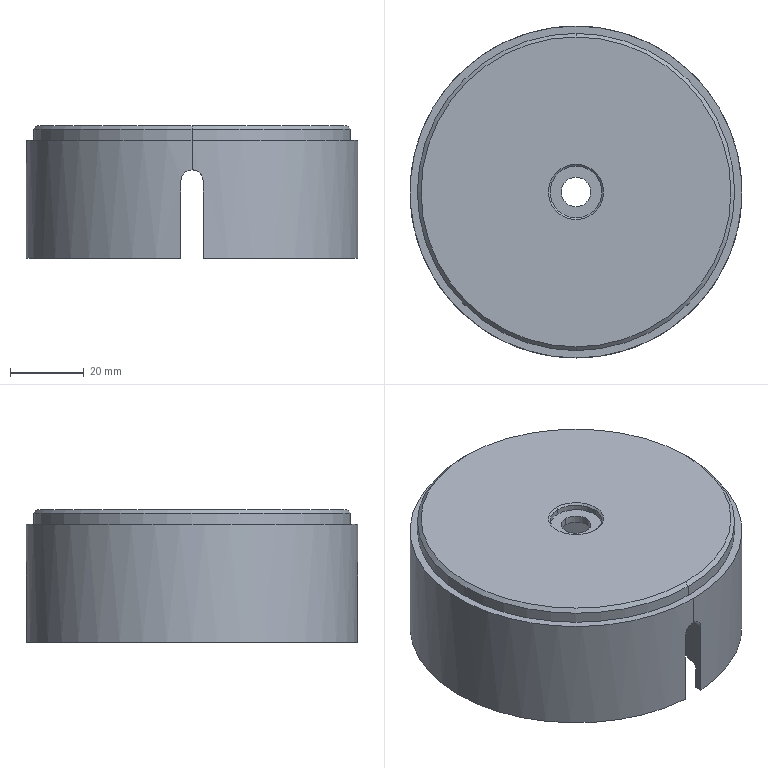Component | SolidWorks | GuideCover-1 | 1 solid | 34 faces | volume 64037 mm3 | cylinder 14 | plane 10 | torus 6 | cone 4 | commonest cylinder face diameters 86 x4 14 x2 90 x2 78 x2 8 x2 6 x2